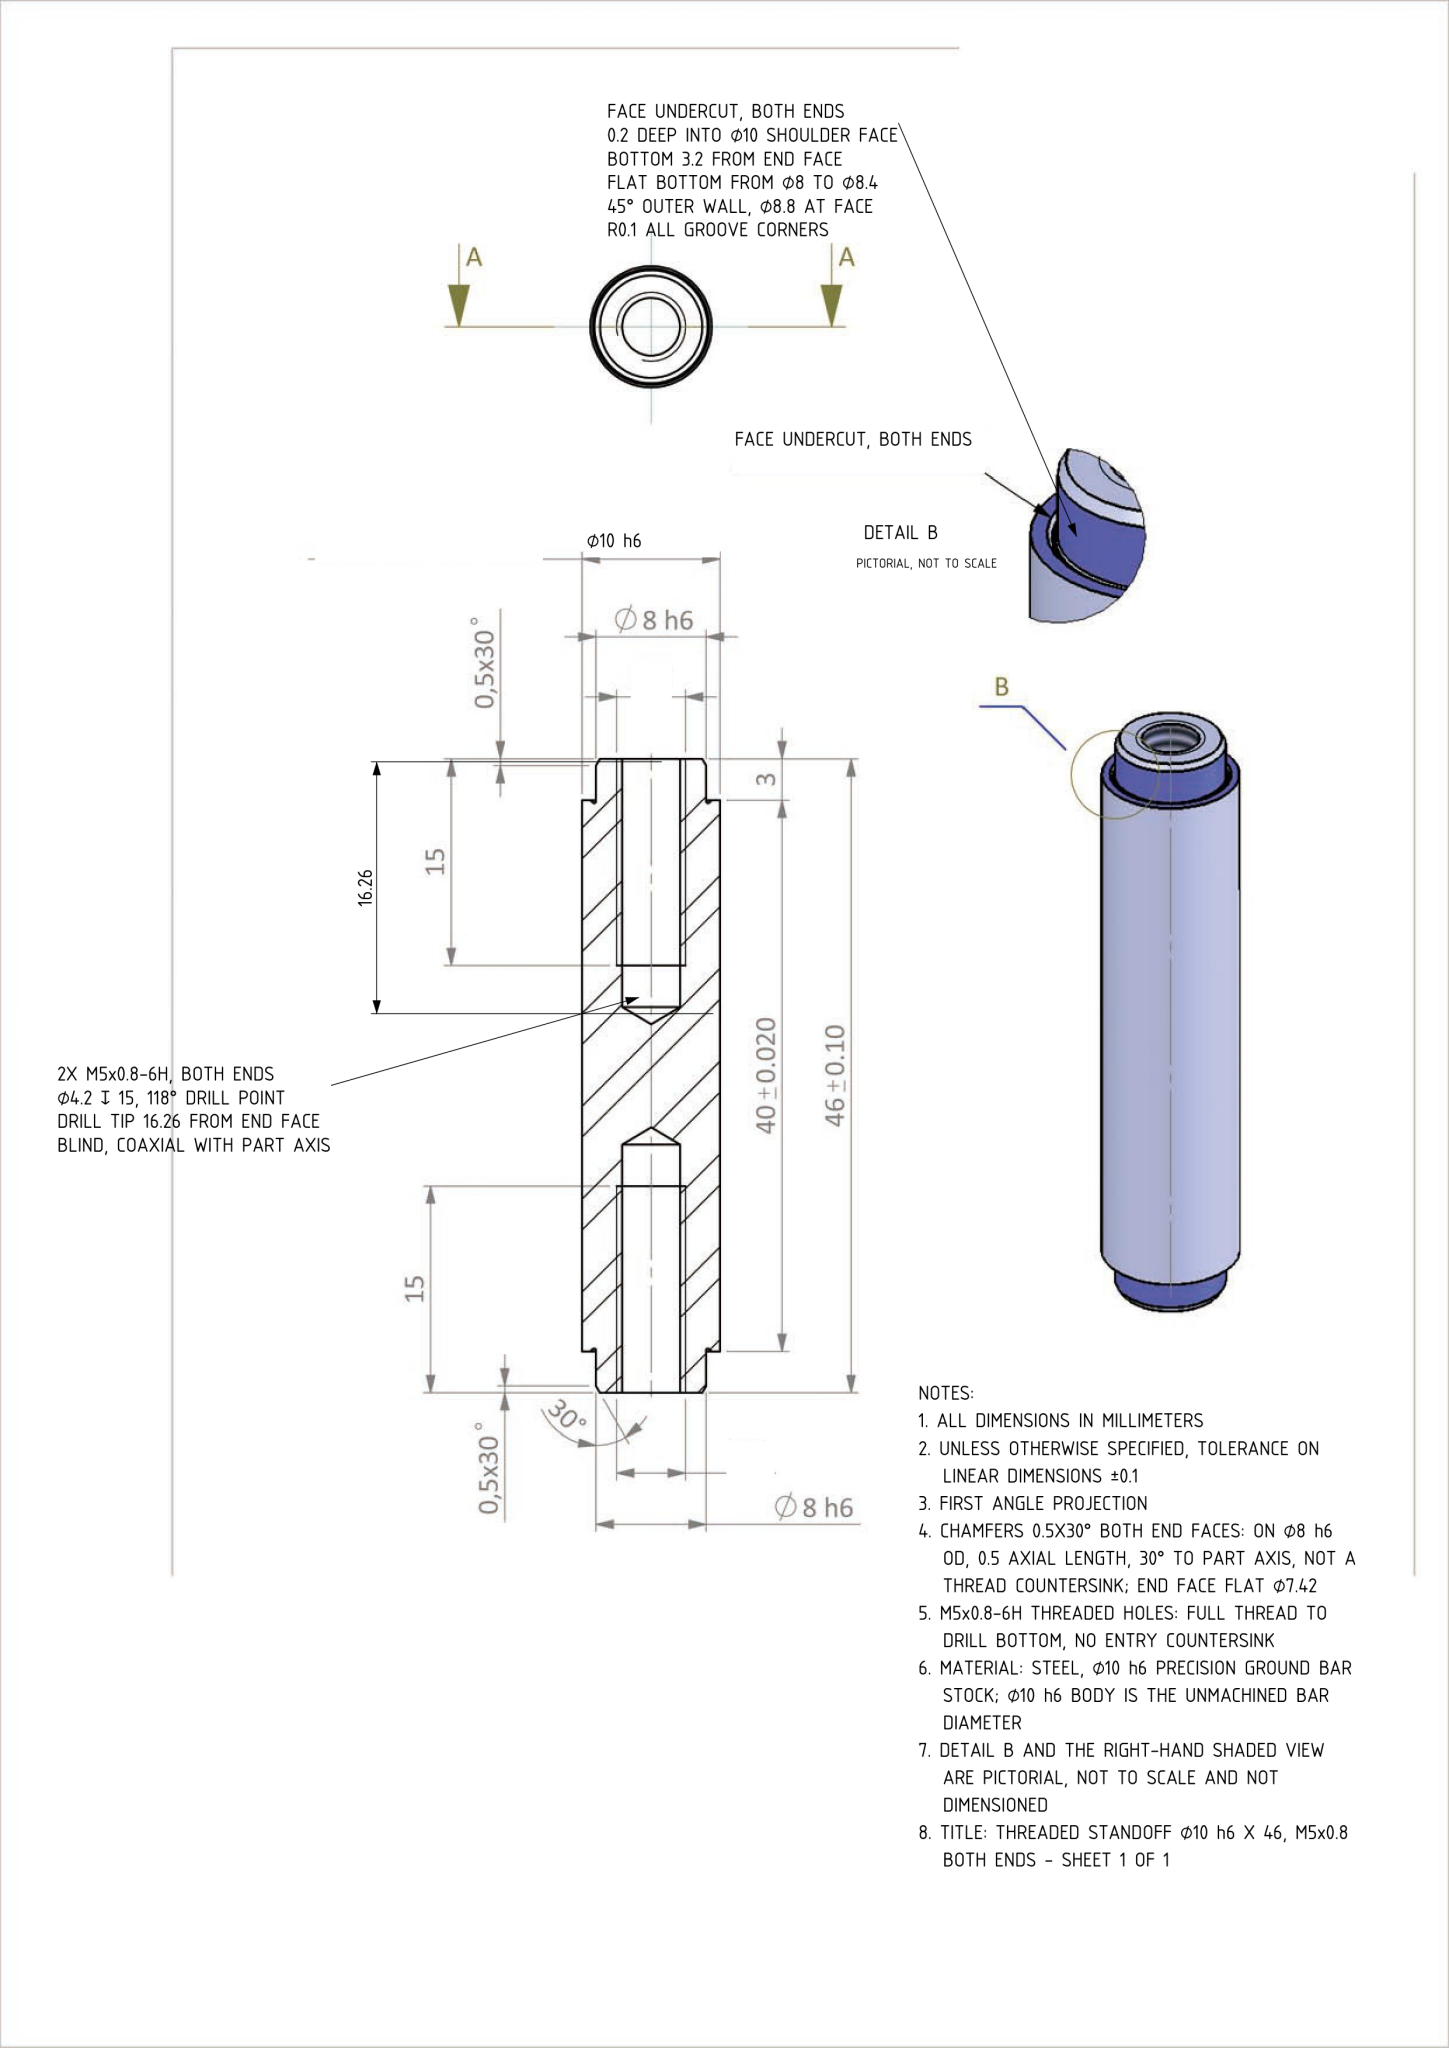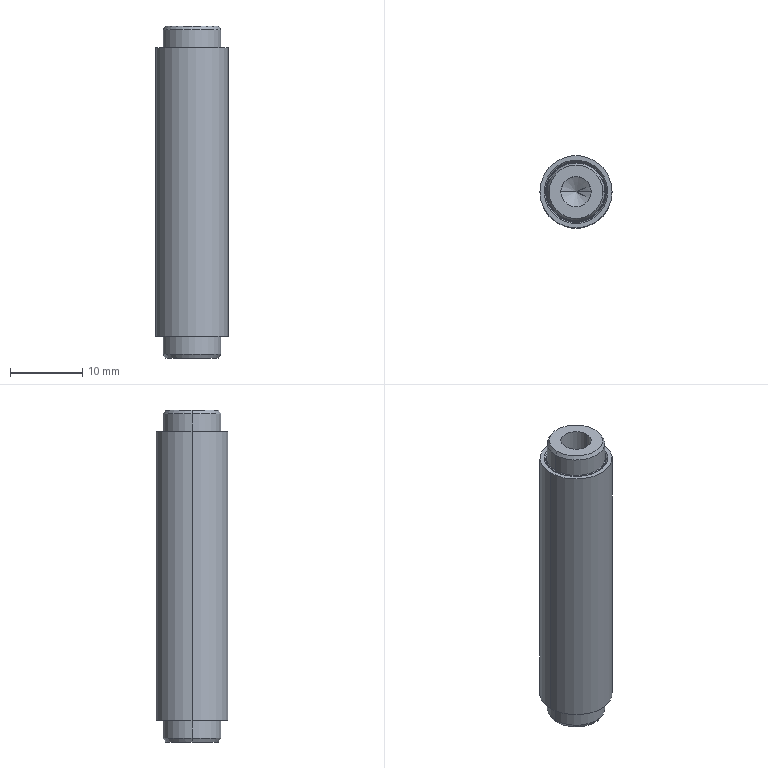Part | NX | mm | 1 solid | 36 faces | box 10 x 10 x 46 mm | volume 2926 mm3 | cone 12 | cylinder 10 | torus 8 | plane 6 | commonest cylinder face diameters 8 x4 4.2 x4 10 x2